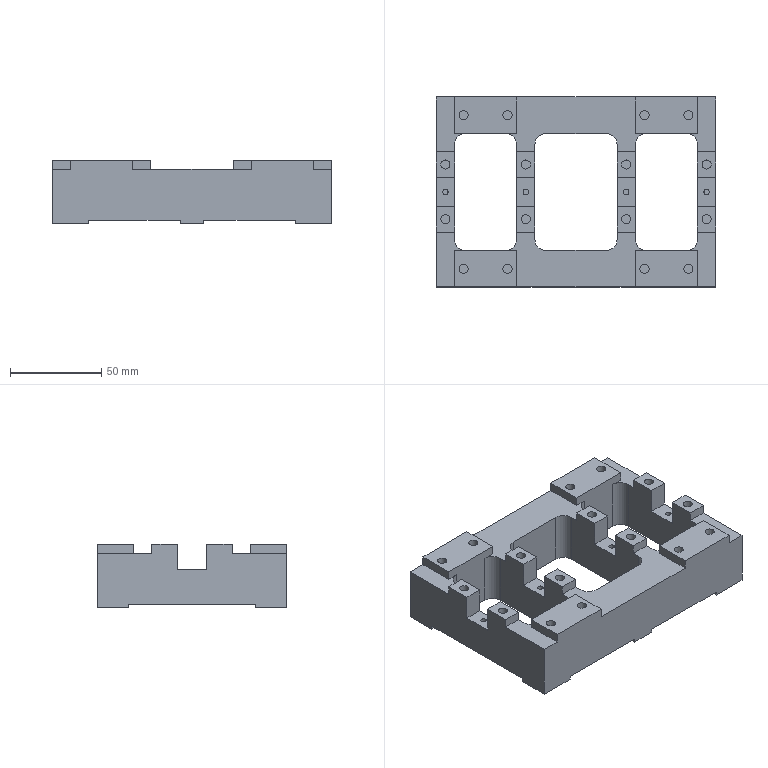Component | NX | 01__27 | 1 solid | 147 faces | volume 257644 mm3 | plane 109 | cylinder 38 | commonest cylinder face diameters 5 x16 12 x12 6 x6 3 x4